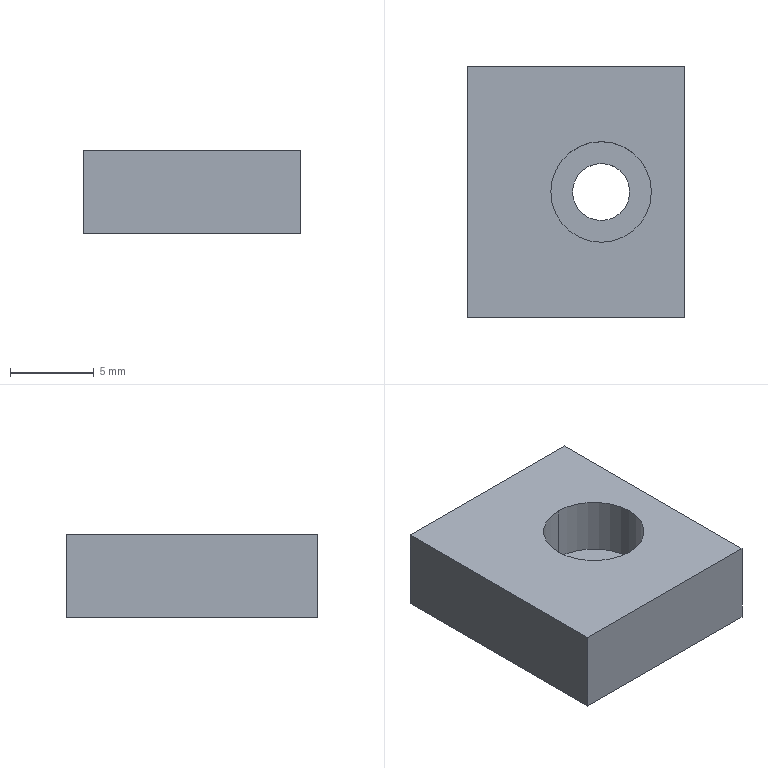Component | SolidWorks | LSDH-4-030-1 | 1 solid | 11 faces | box 13 x 15 x 5 mm | volume 864 mm3 | plane 7 | cylinder 4 | commonest cylinder face diameters 6 x2 3.4 x2
build123d program:
from build123d import *

# Parameters (mm, degrees)
SKETCH1_W                                            = 15
SKETCH1_H                                            = 23
BOSS_EXTRUDE1_DEPTH                                  = 5
HOLE_SIZE_ACCORDING_TO_THE_TYPE_OF_HEX_S_D           = 3.4
HOLE_SIZE_ACCORDING_TO_THE_TYPE_OF_HEX_S_CBORE_D     = 6
HOLE_SIZE_ACCORDING_TO_THE_TYPE_OF_HEX_S_CBORE_DEPTH = 3.4
SKETCH4_W                                            = 15
SKETCH4_H                                            = 10
CUT_EXTRUDE1_DEPTH                                   = 15.612


with BuildPart() as part:
    # Sketch1 → Boss-Extrude1 (new body)
    with BuildSketch(Plane.XY):
        Rectangle(SKETCH1_W, SKETCH1_H)
    extrude(amount=BOSS_EXTRUDE1_DEPTH)

    # Hole size according to the type of hex s (through all)
    with Locations(Plane.XY.offset(5)):
        with Locations((0, 3.5), (0, -6.5)):
            CounterBoreHole(HOLE_SIZE_ACCORDING_TO_THE_TYPE_OF_HEX_S_D / 2, HOLE_SIZE_ACCORDING_TO_THE_TYPE_OF_HEX_S_CBORE_D / 2, HOLE_SIZE_ACCORDING_TO_THE_TYPE_OF_HEX_S_CBORE_DEPTH)

    # Sketch4 → Cut-Extrude1 (cut, through all)
    with BuildSketch(Plane.XY.offset(5)):
        with Locations((0, -6.5)):
            Rectangle(SKETCH4_W, SKETCH4_H)
    extrude(amount=-CUT_EXTRUDE1_DEPTH, mode=Mode.SUBTRACT)


solid = part.part

# Placed as in the assembly
solid = solid.moved(Location((424.805, 375.175, 147.979), (0, 0, 90)))
STEP:
#1=COLOUR_RGB('',0.7922,0.8196,0.9333);
#2=FILL_AREA_STYLE_COLOUR('',#1);
#3=FILL_AREA_STYLE('',(#2));
#4=SURFACE_STYLE_FILL_AREA(#3);
#5=SURFACE_SIDE_STYLE('',(#4));
#6=SURFACE_STYLE_USAGE(.BOTH.,#5);
#7=PRESENTATION_STYLE_ASSIGNMENT((#6));
#8=CARTESIAN_POINT('',(16.587,14.653,5.889));
#9=VERTEX_POINT('',#8);
#10=CARTESIAN_POINT('',(16.587,14.889,5.889));
#11=VERTEX_POINT('',#10);
#12=CARTESIAN_POINT('',(16.587,14.771,5.889));
#13=DIRECTION('',(-0.,0.,1.));
#14=DIRECTION('',(0.,1.,0.));
#15=AXIS2_PLACEMENT_3D('',#12,#13,#14);
#16=CIRCLE('',#15,0.1181);
#17=EDGE_CURVE('',#9,#11,#16,.T.);
#18=ORIENTED_EDGE('',*,*,#17,.F.);
#19=CARTESIAN_POINT('',(16.587,14.653,6.023));
#20=VERTEX_POINT('',#19);
#21=CARTESIAN_POINT('',(16.587,14.653,6.023));
#22=DIRECTION('',(-0.,0.,1.));
#23=VECTOR('',#22,39.37);
#24=LINE('',#21,#23);
#25=EDGE_CURVE('',#9,#20,#24,.T.);
#26=ORIENTED_EDGE('',*,*,#25,.T.);
#27=CARTESIAN_POINT('',(16.587,14.889,6.023));
#28=VERTEX_POINT('',#27);
#29=CARTESIAN_POINT('',(16.587,14.771,6.023));
#30=DIRECTION('',(-0.,0.,1.));
#31=DIRECTION('',(0.,1.,0.));
#32=AXIS2_PLACEMENT_3D('',#29,#30,#31);
#33=CIRCLE('',#32,0.1181);
#34=EDGE_CURVE('',#20,#28,#33,.T.);
#35=ORIENTED_EDGE('',*,*,#34,.T.);
#36=CARTESIAN_POINT('',(16.587,14.889,6.023));
#37=DIRECTION('',(-0.,0.,1.));
#38=VECTOR('',#37,39.37);
#39=LINE('',#36,#38);
#40=EDGE_CURVE('',#11,#28,#39,.T.);
#41=ORIENTED_EDGE('',*,*,#40,.F.);
#42=EDGE_LOOP('',(#18,#26,#35,#41));
#43=FACE_OUTER_BOUND('',#42,.T.);
#44=CARTESIAN_POINT('',(16.587,14.771,6.023));
#45=DIRECTION('',(-0.,0.,1.));
#46=DIRECTION('',(0.,1.,0.));
#47=AXIS2_PLACEMENT_3D('',#44,#45,#46);
#48=CYLINDRICAL_SURFACE('',#47,0.1181);
#49=ADVANCED_FACE('',(#43),#48,.F.);
#50=CARTESIAN_POINT('',(16.587,14.704,5.826));
#51=VERTEX_POINT('',#50);
#52=CARTESIAN_POINT('',(16.587,14.838,5.826));
#53=VERTEX_POINT('',#52);
#54=CARTESIAN_POINT('',(16.587,14.771,5.826));
#55=DIRECTION('',(-0.,0.,1.));
#56=DIRECTION('',(0.,1.,0.));
#57=AXIS2_PLACEMENT_3D('',#54,#55,#56);
#58=CIRCLE('',#57,0.06693);
#59=EDGE_CURVE('',#51,#53,#58,.T.);
#60=ORIENTED_EDGE('',*,*,#59,.F.);
#61=CARTESIAN_POINT('',(16.587,14.704,5.889));
#62=VERTEX_POINT('',#61);
#63=CARTESIAN_POINT('',(16.587,14.704,6.023));
#64=DIRECTION('',(-0.,0.,1.));
#65=VECTOR('',#64,39.37);
#66=LINE('',#63,#65);
#67=EDGE_CURVE('',#51,#62,#66,.T.);
#68=ORIENTED_EDGE('',*,*,#67,.T.);
#69=CARTESIAN_POINT('',(16.587,14.838,5.889));
#70=VERTEX_POINT('',#69);
#71=CARTESIAN_POINT('',(16.587,14.771,5.889));
#72=DIRECTION('',(-0.,0.,1.));
#73=DIRECTION('',(0.,1.,0.));
#74=AXIS2_PLACEMENT_3D('',#71,#72,#73);
#75=CIRCLE('',#74,0.06693);
#76=EDGE_CURVE('',#62,#70,#75,.T.);
#77=ORIENTED_EDGE('',*,*,#76,.T.);
#78=CARTESIAN_POINT('',(16.587,14.838,6.023));
#79=DIRECTION('',(-0.,0.,1.));
#80=VECTOR('',#79,39.37);
#81=LINE('',#78,#80);
#82=EDGE_CURVE('',#53,#70,#81,.T.);
#83=ORIENTED_EDGE('',*,*,#82,.F.);
#84=EDGE_LOOP('',(#60,#68,#77,#83));
#85=FACE_OUTER_BOUND('',#84,.T.);
#86=CARTESIAN_POINT('',(16.587,14.771,6.023));
#87=DIRECTION('',(-0.,0.,1.));
#88=DIRECTION('',(0.,1.,0.));
#89=AXIS2_PLACEMENT_3D('',#86,#87,#88);
#90=CYLINDRICAL_SURFACE('',#89,0.06693);
#91=ADVANCED_FACE('',(#85),#90,.F.);
#92=CARTESIAN_POINT('',(16.784,15.066,6.023));
#93=VERTEX_POINT('',#92);
#94=CARTESIAN_POINT('',(16.272,15.066,6.023));
#95=VERTEX_POINT('',#94);
#96=CARTESIAN_POINT('',(16.272,15.066,6.023));
#97=DIRECTION('',(-1.,-0.,-0.));
#98=VECTOR('',#97,39.37);
#99=LINE('',#96,#98);
#100=EDGE_CURVE('',#93,#95,#99,.T.);
#101=ORIENTED_EDGE('',*,*,#100,.F.);
#102=CARTESIAN_POINT('',(16.784,15.066,5.826));
#103=VERTEX_POINT('',#102);
#104=CARTESIAN_POINT('',(16.784,15.066,5.826));
#105=DIRECTION('',(-0.,0.,1.));
#106=VECTOR('',#105,39.37);
#107=LINE('',#104,#106);
#108=EDGE_CURVE('',#103,#93,#107,.T.);
#109=ORIENTED_EDGE('',*,*,#108,.F.);
#110=CARTESIAN_POINT('',(16.272,15.066,5.826));
#111=VERTEX_POINT('',#110);
#112=CARTESIAN_POINT('',(16.272,15.066,5.826));
#113=DIRECTION('',(-1.,-0.,-0.));
#114=VECTOR('',#113,39.37);
#115=LINE('',#112,#114);
#116=EDGE_CURVE('',#103,#111,#115,.T.);
#117=ORIENTED_EDGE('',*,*,#116,.T.);
#118=CARTESIAN_POINT('',(16.272,15.066,6.023));
#119=DIRECTION('',(0.,-0.,-1.));
#120=VECTOR('',#119,39.37);
#121=LINE('',#118,#120);
#122=EDGE_CURVE('',#95,#111,#121,.T.);
#123=ORIENTED_EDGE('',*,*,#122,.F.);
#124=EDGE_LOOP('',(#101,#109,#117,#123));
#125=FACE_OUTER_BOUND('',#124,.T.);
#126=CARTESIAN_POINT('',(16.272,15.066,6.023));
#127=DIRECTION('',(0.,-1.,0.));
#128=DIRECTION('',(1.,0.,0.));
#129=AXIS2_PLACEMENT_3D('',#126,#127,#128);
#130=PLANE('',#129);
#131=ADVANCED_FACE('',(#125),#130,.F.);
#132=CARTESIAN_POINT('',(16.272,14.475,5.826));
#133=VERTEX_POINT('',#132);
#134=CARTESIAN_POINT('',(16.272,14.475,5.826));
#135=DIRECTION('',(0.,-1.,0.));
#136=VECTOR('',#135,39.37);
#137=LINE('',#134,#136);
#138=EDGE_CURVE('',#111,#133,#137,.T.);
#139=ORIENTED_EDGE('',*,*,#138,.T.);
#140=CARTESIAN_POINT('',(16.272,14.475,6.023));
#141=VERTEX_POINT('',#140);
#142=CARTESIAN_POINT('',(16.272,14.475,6.023));
#143=DIRECTION('',(0.,-0.,-1.));
#144=VECTOR('',#143,39.37);
#145=LINE('',#142,#144);
#146=EDGE_CURVE('',#141,#133,#145,.T.);
#147=ORIENTED_EDGE('',*,*,#146,.F.);
#148=CARTESIAN_POINT('',(16.272,14.475,6.023));
#149=DIRECTION('',(0.,-1.,0.));
#150=VECTOR('',#149,39.37);
#151=LINE('',#148,#150);
#152=EDGE_CURVE('',#95,#141,#151,.T.);
#153=ORIENTED_EDGE('',*,*,#152,.F.);
#154=ORIENTED_EDGE('',*,*,#122,.T.);
#155=EDGE_LOOP('',(#139,#147,#153,#154));
#156=FACE_OUTER_BOUND('',#155,.T.);
#157=CARTESIAN_POINT('',(16.272,14.475,6.023));
#158=DIRECTION('',(1.,0.,0.));
#159=DIRECTION('',(0.,-0.,-1.));
#160=AXIS2_PLACEMENT_3D('',#157,#158,#159);
#161=PLANE('',#160);
#162=ADVANCED_FACE('',(#156),#161,.F.);
#163=CARTESIAN_POINT('',(16.784,14.475,5.826));
#164=VERTEX_POINT('',#163);
#165=CARTESIAN_POINT('',(16.272,14.475,5.826));
#166=DIRECTION('',(1.,0.,0.));
#167=VECTOR('',#166,39.37);
#168=LINE('',#165,#167);
#169=EDGE_CURVE('',#133,#164,#168,.T.);
#170=ORIENTED_EDGE('',*,*,#169,.T.);
#171=CARTESIAN_POINT('',(16.784,14.475,6.023));
#172=VERTEX_POINT('',#171);
#173=CARTESIAN_POINT('',(16.784,14.475,5.826));
#174=DIRECTION('',(-0.,0.,1.));
#175=VECTOR('',#174,39.37);
#176=LINE('',#173,#175);
#177=EDGE_CURVE('',#164,#172,#176,.T.);
#178=ORIENTED_EDGE('',*,*,#177,.T.);
#179=CARTESIAN_POINT('',(16.272,14.475,6.023));
#180=DIRECTION('',(1.,0.,0.));
#181=VECTOR('',#180,39.37);
#182=LINE('',#179,#181);
#183=EDGE_CURVE('',#141,#172,#182,.T.);
#184=ORIENTED_EDGE('',*,*,#183,.F.);
#185=ORIENTED_EDGE('',*,*,#146,.T.);
#186=EDGE_LOOP('',(#170,#178,#184,#185));
#187=FACE_OUTER_BOUND('',#186,.T.);
#188=CARTESIAN_POINT('',(16.272,14.475,6.023));
#189=DIRECTION('',(-0.,1.,-0.));
#190=DIRECTION('',(-1.,-0.,-0.));
#191=AXIS2_PLACEMENT_3D('',#188,#189,#190);
#192=PLANE('',#191);
#193=ADVANCED_FACE('',(#187),#192,.F.);
#194=CARTESIAN_POINT('',(16.784,14.475,6.023));
#195=DIRECTION('',(0.,-1.,0.));
#196=VECTOR('',#195,39.37);
#197=LINE('',#194,#196);
#198=EDGE_CURVE('',#93,#172,#197,.T.);
#199=ORIENTED_EDGE('',*,*,#198,.F.);
#200=ORIENTED_EDGE('',*,*,#100,.T.);
#201=ORIENTED_EDGE('',*,*,#152,.T.);
#202=ORIENTED_EDGE('',*,*,#183,.T.);
#203=EDGE_LOOP('',(#199,#200,#201,#202));
#204=FACE_OUTER_BOUND('',#203,.T.);
#205=CARTESIAN_POINT('',(16.587,14.771,6.023));
#206=DIRECTION('',(-0.,0.,1.));
#207=DIRECTION('',(0.,1.,0.));
#208=AXIS2_PLACEMENT_3D('',#205,#206,#207);
#209=CIRCLE('',#208,0.1181);
#210=EDGE_CURVE('',#28,#20,#209,.T.);
#211=ORIENTED_EDGE('',*,*,#210,.F.);
#212=ORIENTED_EDGE('',*,*,#34,.F.);
#213=EDGE_LOOP('',(#211,#212));
#214=FACE_BOUND('',#213,.T.);
#215=CARTESIAN_POINT('',(16.725,14.771,6.023));
#216=DIRECTION('',(-0.,0.,1.));
#217=DIRECTION('',(0.,1.,-0.));
#218=AXIS2_PLACEMENT_3D('',#215,#216,#217);
#219=PLANE('',#218);
#220=ADVANCED_FACE('',(#204,#214),#219,.T.);
#221=CARTESIAN_POINT('',(16.587,14.771,5.826));
#222=DIRECTION('',(-0.,0.,1.));
#223=DIRECTION('',(0.,1.,0.));
#224=AXIS2_PLACEMENT_3D('',#221,#222,#223);
#225=CIRCLE('',#224,0.06693);
#226=EDGE_CURVE('',#53,#51,#225,.T.);
#227=ORIENTED_EDGE('',*,*,#226,.T.);
#228=ORIENTED_EDGE('',*,*,#59,.T.);
#229=EDGE_LOOP('',(#227,#228));
#230=FACE_BOUND('',#229,.T.);
#231=ORIENTED_EDGE('',*,*,#116,.F.);
#232=CARTESIAN_POINT('',(16.784,14.475,5.826));
#233=DIRECTION('',(0.,-1.,0.));
#234=VECTOR('',#233,39.37);
#235=LINE('',#232,#234);
#236=EDGE_CURVE('',#103,#164,#235,.T.);
#237=ORIENTED_EDGE('',*,*,#236,.T.);
#238=ORIENTED_EDGE('',*,*,#169,.F.);
#239=ORIENTED_EDGE('',*,*,#138,.F.);
#240=EDGE_LOOP('',(#231,#237,#238,#239));
#241=FACE_OUTER_BOUND('',#240,.T.);
#242=CARTESIAN_POINT('',(16.725,14.771,5.826));
#243=DIRECTION('',(-0.,0.,1.));
#244=DIRECTION('',(0.,1.,-0.));
#245=AXIS2_PLACEMENT_3D('',#242,#243,#244);
#246=PLANE('',#245);
#247=ADVANCED_FACE('',(#230,#241),#246,.F.);
#248=ORIENTED_EDGE('',*,*,#67,.F.);
#249=ORIENTED_EDGE('',*,*,#226,.F.);
#250=ORIENTED_EDGE('',*,*,#82,.T.);
#251=CARTESIAN_POINT('',(16.587,14.771,5.889));
#252=DIRECTION('',(-0.,0.,1.));
#253=DIRECTION('',(0.,1.,0.));
#254=AXIS2_PLACEMENT_3D('',#251,#252,#253);
#255=CIRCLE('',#254,0.06693);
#256=EDGE_CURVE('',#70,#62,#255,.T.);
#257=ORIENTED_EDGE('',*,*,#256,.T.);
#258=EDGE_LOOP('',(#248,#249,#250,#257));
#259=FACE_OUTER_BOUND('',#258,.T.);
#260=CARTESIAN_POINT('',(16.587,14.771,6.023));
#261=DIRECTION('',(-0.,0.,1.));
#262=DIRECTION('',(0.,1.,0.));
#263=AXIS2_PLACEMENT_3D('',#260,#261,#262);
#264=CYLINDRICAL_SURFACE('',#263,0.06693);
#265=ADVANCED_FACE('',(#259),#264,.F.);
#266=ORIENTED_EDGE('',*,*,#256,.F.);
#267=ORIENTED_EDGE('',*,*,#76,.F.);
#268=EDGE_LOOP('',(#266,#267));
#269=FACE_BOUND('',#268,.T.);
#270=CARTESIAN_POINT('',(16.587,14.771,5.889));
#271=DIRECTION('',(-0.,0.,1.));
#272=DIRECTION('',(0.,1.,0.));
#273=AXIS2_PLACEMENT_3D('',#270,#271,#272);
#274=CIRCLE('',#273,0.1181);
#275=EDGE_CURVE('',#11,#9,#274,.T.);
#276=ORIENTED_EDGE('',*,*,#275,.T.);
#277=ORIENTED_EDGE('',*,*,#17,.T.);
#278=EDGE_LOOP('',(#276,#277));
#279=FACE_OUTER_BOUND('',#278,.T.);
#280=CARTESIAN_POINT('',(16.587,14.838,5.889));
#281=DIRECTION('',(0.,-0.,-1.));
#282=DIRECTION('',(0.,-1.,0.));
#283=AXIS2_PLACEMENT_3D('',#280,#281,#282);
#284=PLANE('',#283);
#285=ADVANCED_FACE('',(#269,#279),#284,.F.);
#286=ORIENTED_EDGE('',*,*,#25,.F.);
#287=ORIENTED_EDGE('',*,*,#275,.F.);
#288=ORIENTED_EDGE('',*,*,#40,.T.);
#289=ORIENTED_EDGE('',*,*,#210,.T.);
#290=EDGE_LOOP('',(#286,#287,#288,#289));
#291=FACE_OUTER_BOUND('',#290,.T.);
#292=CARTESIAN_POINT('',(16.587,14.771,6.023));
#293=DIRECTION('',(-0.,0.,1.));
#294=DIRECTION('',(0.,1.,0.));
#295=AXIS2_PLACEMENT_3D('',#292,#293,#294);
#296=CYLINDRICAL_SURFACE('',#295,0.1181);
#297=ADVANCED_FACE('',(#291),#296,.F.);
#298=ORIENTED_EDGE('',*,*,#198,.T.);
#299=ORIENTED_EDGE('',*,*,#177,.F.);
#300=ORIENTED_EDGE('',*,*,#236,.F.);
#301=ORIENTED_EDGE('',*,*,#108,.T.);
#302=EDGE_LOOP('',(#298,#299,#300,#301));
#303=FACE_OUTER_BOUND('',#302,.T.);
#304=CARTESIAN_POINT('',(16.784,14.475,5.826));
#305=DIRECTION('',(-1.,-0.,-0.));
#306=DIRECTION('',(-0.,0.,1.));
#307=AXIS2_PLACEMENT_3D('',#304,#305,#306);
#308=PLANE('',#307);
#309=ADVANCED_FACE('',(#303),#308,.F.);
#310=CLOSED_SHELL('',(#49,#91,#131,#162,#193,#220,#247,#265,#285,#297,#309));
#311=MANIFOLD_SOLID_BREP('',#310);
#312=STYLED_ITEM('',(#7),#311);
#313=PRESENTATION_LAYER_ASSIGNMENT('','',(#312));
#314=(LENGTH_UNIT()NAMED_UNIT(*)SI_UNIT($,.METRE.));
#315=LENGTH_MEASURE_WITH_UNIT(LENGTH_MEASURE(0.0254),#314);
#316=DIMENSIONAL_EXPONENTS(1.,0.,0.,0.,0.,0.,0.);
#317=(CONVERSION_BASED_UNIT('',#315)LENGTH_UNIT()NAMED_UNIT(#316));
#318=UNCERTAINTY_MEASURE_WITH_UNIT(LENGTH_MEASURE(0.00001),#317,'','');
#319=(NAMED_UNIT(*)PLANE_ANGLE_UNIT()SI_UNIT($,.RADIAN.));
#320=(NAMED_UNIT(*)SI_UNIT($,.STERADIAN.)SOLID_ANGLE_UNIT());
#321=(GEOMETRIC_REPRESENTATION_CONTEXT(3)GLOBAL_UNCERTAINTY_ASSIGNED_CONTEXT((#318))GLOBAL_UNIT_ASSIGNED_CONTEXT((#317,#319,#320))REPRESENTATION_CONTEXT('',''));
#322=MECHANICAL_DESIGN_GEOMETRIC_PRESENTATION_REPRESENTATION('',(#312),#321);
#323=CARTESIAN_POINT('',(0.,0.,0.));
#324=DIRECTION('',(0.,0.,1.));
#325=DIRECTION('',(1.,0.,0.));
#326=AXIS2_PLACEMENT_3D('',#323,#324,#325);
#327=(LENGTH_UNIT()NAMED_UNIT(*)SI_UNIT($,.METRE.));
#328=LENGTH_MEASURE_WITH_UNIT(LENGTH_MEASURE(0.0254),#327);
#329=DIMENSIONAL_EXPONENTS(1.,0.,0.,0.,0.,0.,0.);
#330=(CONVERSION_BASED_UNIT('',#328)LENGTH_UNIT()NAMED_UNIT(#329));
#331=UNCERTAINTY_MEASURE_WITH_UNIT(LENGTH_MEASURE(0.00001),#330,'','');
#332=(NAMED_UNIT(*)PLANE_ANGLE_UNIT()SI_UNIT($,.RADIAN.));
#333=(NAMED_UNIT(*)SI_UNIT($,.STERADIAN.)SOLID_ANGLE_UNIT());
#334=(GEOMETRIC_REPRESENTATION_CONTEXT(3)GLOBAL_UNCERTAINTY_ASSIGNED_CONTEXT((#331))GLOBAL_UNIT_ASSIGNED_CONTEXT((#330,#332,#333))REPRESENTATION_CONTEXT('',''));
#335=ADVANCED_BREP_SHAPE_REPRESENTATION('',(#311,#326),#334);